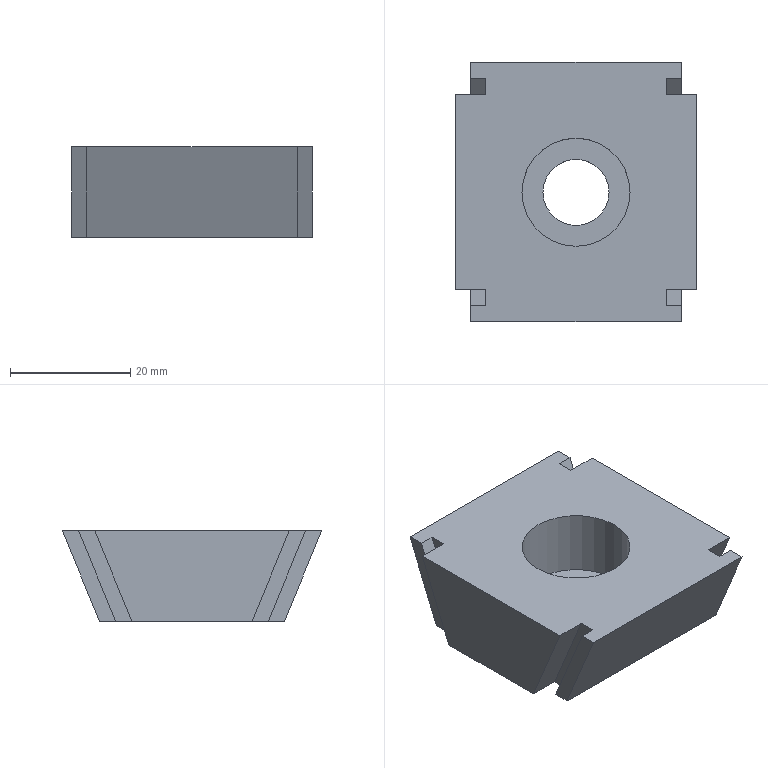Component | NX | MOVING_SLIDER_2 | 1 solid | 25 faces | volume 17814 mm3 | plane 23 | cylinder 2 | commonest cylinder face diameters 11 x1 18 x1